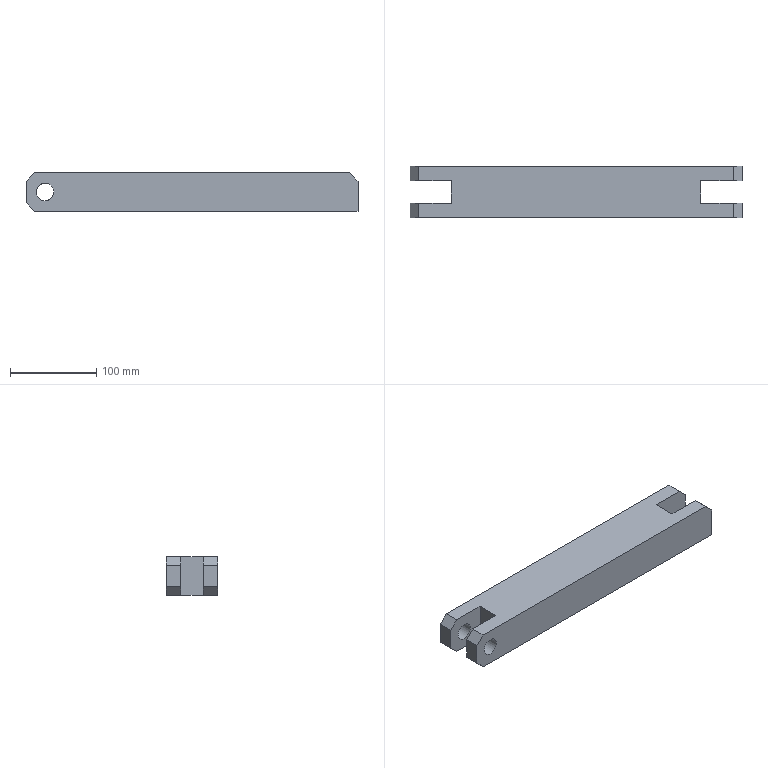Component | NX | CLAMP_PLATE | 1 solid | 22 faces | volume 908699 mm3 | plane 20 | cylinder 2 | commonest cylinder face diameters 20 x2